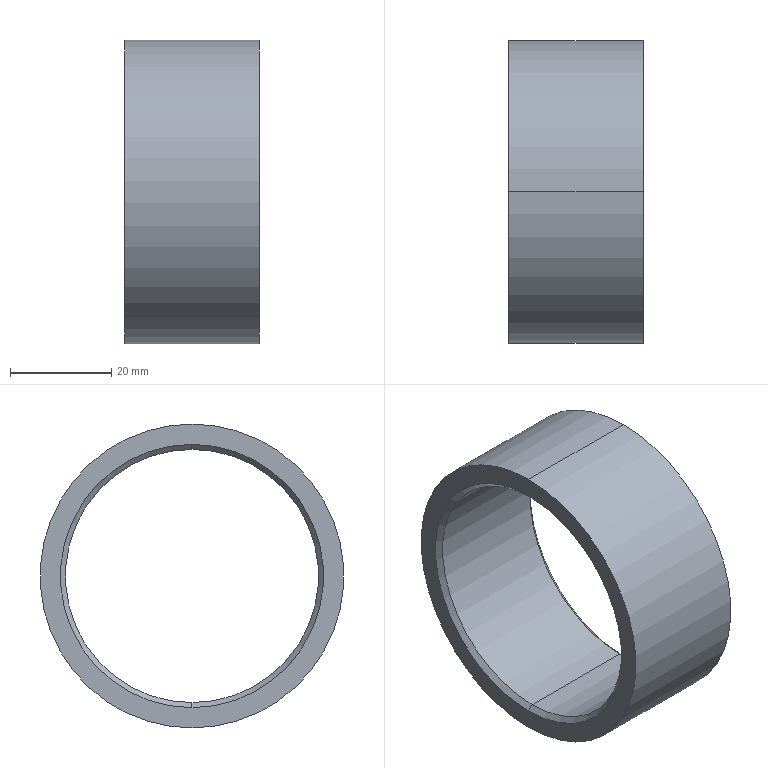Component | SolidWorks | SpindleSleeve4-1 | 1 solid | 10 faces | box 26.5 x 60 x 60 mm | volume 22735 mm3 | cone 4 | cylinder 4 | plane 2 | commonest cylinder face diameters 50 x2 60 x2
build123d program:
from build123d import *

# Parameters (mm, degrees)
SKETCH1_R           = 30
SKETCH1_R_2         = 25
BOSS_EXTRUDE1_DEPTH = 13.25
CHAMFER1_SIZE       = 1


with BuildPart() as part:
    # Sketch1 → Boss-Extrude1 (new, symmetric)
    with BuildSketch(Plane(origin=(0, 0, 0), x_dir=(0, 0, -1), z_dir=(1, 0, 0))):
        Circle(SKETCH1_R)
        Circle(SKETCH1_R_2, mode=Mode.SUBTRACT)
    extrude(amount=BOSS_EXTRUDE1_DEPTH, both=True)

    # Chamfer1
    chamfer1_edges = [part.edges().sort_by_distance(p)[0] for p in [
        (-13.25, 0, 25),
        (13.25, 0, 25),
    ]]
    chamfer(chamfer1_edges, length=CHAMFER1_SIZE)


solid = part.part

# Placed as in the assembly
solid = solid.moved(Location((-804.447, 34.532, 0), (0, 0, 0)))
STEP:
#1=COLOUR_RGB('',0.7922,0.8196,0.9333);
#2=FILL_AREA_STYLE_COLOUR('',#1);
#3=FILL_AREA_STYLE('',(#2));
#4=SURFACE_STYLE_FILL_AREA(#3);
#5=SURFACE_SIDE_STYLE('',(#4));
#6=SURFACE_STYLE_USAGE(.BOTH.,#5);
#7=PRESENTATION_STYLE_ASSIGNMENT((#6));
#8=CARTESIAN_POINT('',(-31.189,1.36,0.9843));
#9=VERTEX_POINT('',#8);
#10=CARTESIAN_POINT('',(-31.189,1.36,-0.9843));
#11=VERTEX_POINT('',#10);
#12=CARTESIAN_POINT('',(-31.189,1.36,0.));
#13=DIRECTION('',(1.,0.,0.));
#14=DIRECTION('',(0.,0.,-1.));
#15=AXIS2_PLACEMENT_3D('',#12,#13,#14);
#16=CIRCLE('',#15,0.9843);
#17=EDGE_CURVE('',#9,#11,#16,.T.);
#18=ORIENTED_EDGE('',*,*,#17,.F.);
#19=CARTESIAN_POINT('',(-31.149,1.36,1.024));
#20=VERTEX_POINT('',#19);
#21=CARTESIAN_POINT('',(-31.189,1.36,0.9843));
#22=DIRECTION('',(0.7071,0.,0.7071));
#23=VECTOR('',#22,39.37);
#24=LINE('',#21,#23);
#25=EDGE_CURVE('',#9,#20,#24,.T.);
#26=ORIENTED_EDGE('',*,*,#25,.T.);
#27=CARTESIAN_POINT('',(-31.149,1.36,-1.024));
#28=VERTEX_POINT('',#27);
#29=CARTESIAN_POINT('',(-31.149,1.36,0.));
#30=DIRECTION('',(-1.,0.,0.));
#31=DIRECTION('',(0.,0.,-1.));
#32=AXIS2_PLACEMENT_3D('',#29,#30,#31);
#33=CIRCLE('',#32,1.024);
#34=EDGE_CURVE('',#28,#20,#33,.T.);
#35=ORIENTED_EDGE('',*,*,#34,.F.);
#36=CARTESIAN_POINT('',(-31.189,1.36,-0.9843));
#37=DIRECTION('',(0.7071,0.,-0.7071));
#38=VECTOR('',#37,39.37);
#39=LINE('',#36,#38);
#40=EDGE_CURVE('',#11,#28,#39,.T.);
#41=ORIENTED_EDGE('',*,*,#40,.F.);
#42=EDGE_LOOP('',(#18,#26,#35,#41));
#43=FACE_OUTER_BOUND('',#42,.T.);
#44=CARTESIAN_POINT('',(-31.189,1.36,0.));
#45=DIRECTION('',(1.,0.,0.));
#46=DIRECTION('',(0.,0.,-1.));
#47=AXIS2_PLACEMENT_3D('',#44,#45,#46);
#48=CONICAL_SURFACE('',#47,0.9843,0.7854);
#49=ADVANCED_FACE('',(#43),#48,.F.);
#50=CARTESIAN_POINT('',(-32.153,1.36,-0.9843));
#51=VERTEX_POINT('',#50);
#52=CARTESIAN_POINT('',(-32.153,1.36,0.9843));
#53=VERTEX_POINT('',#52);
#54=CARTESIAN_POINT('',(-32.153,1.36,0.));
#55=DIRECTION('',(-1.,0.,0.));
#56=DIRECTION('',(0.,0.,-1.));
#57=AXIS2_PLACEMENT_3D('',#54,#55,#56);
#58=CIRCLE('',#57,0.9843);
#59=EDGE_CURVE('',#51,#53,#58,.T.);
#60=ORIENTED_EDGE('',*,*,#59,.F.);
#61=CARTESIAN_POINT('',(-32.193,1.36,-1.024));
#62=VERTEX_POINT('',#61);
#63=CARTESIAN_POINT('',(-32.193,1.36,-1.024));
#64=DIRECTION('',(-0.7071,0.,-0.7071));
#65=VECTOR('',#64,39.37);
#66=LINE('',#63,#65);
#67=EDGE_CURVE('',#51,#62,#66,.T.);
#68=ORIENTED_EDGE('',*,*,#67,.T.);
#69=CARTESIAN_POINT('',(-32.193,1.36,1.024));
#70=VERTEX_POINT('',#69);
#71=CARTESIAN_POINT('',(-32.193,1.36,0.));
#72=DIRECTION('',(1.,0.,0.));
#73=DIRECTION('',(0.,0.,-1.));
#74=AXIS2_PLACEMENT_3D('',#71,#72,#73);
#75=CIRCLE('',#74,1.024);
#76=EDGE_CURVE('',#70,#62,#75,.T.);
#77=ORIENTED_EDGE('',*,*,#76,.F.);
#78=CARTESIAN_POINT('',(-32.193,1.36,1.024));
#79=DIRECTION('',(-0.7071,0.,0.7071));
#80=VECTOR('',#79,39.37);
#81=LINE('',#78,#80);
#82=EDGE_CURVE('',#53,#70,#81,.T.);
#83=ORIENTED_EDGE('',*,*,#82,.F.);
#84=EDGE_LOOP('',(#60,#68,#77,#83));
#85=FACE_OUTER_BOUND('',#84,.T.);
#86=CARTESIAN_POINT('',(-32.193,1.36,0.));
#87=DIRECTION('',(-1.,0.,0.));
#88=DIRECTION('',(0.,0.,1.));
#89=AXIS2_PLACEMENT_3D('',#86,#87,#88);
#90=CONICAL_SURFACE('',#89,1.024,0.7854);
#91=ADVANCED_FACE('',(#85),#90,.F.);
#92=ORIENTED_EDGE('',*,*,#17,.T.);
#93=CARTESIAN_POINT('',(-31.149,1.36,-0.9843));
#94=DIRECTION('',(-1.,0.,0.));
#95=VECTOR('',#94,39.37);
#96=LINE('',#93,#95);
#97=EDGE_CURVE('',#11,#51,#96,.T.);
#98=ORIENTED_EDGE('',*,*,#97,.T.);
#99=ORIENTED_EDGE('',*,*,#59,.T.);
#100=CARTESIAN_POINT('',(-31.149,1.36,0.9843));
#101=DIRECTION('',(-1.,0.,0.));
#102=VECTOR('',#101,39.37);
#103=LINE('',#100,#102);
#104=EDGE_CURVE('',#9,#53,#103,.T.);
#105=ORIENTED_EDGE('',*,*,#104,.F.);
#106=EDGE_LOOP('',(#92,#98,#99,#105));
#107=FACE_OUTER_BOUND('',#106,.T.);
#108=CARTESIAN_POINT('',(-31.149,1.36,0.));
#109=DIRECTION('',(-1.,0.,0.));
#110=DIRECTION('',(0.,0.,1.));
#111=AXIS2_PLACEMENT_3D('',#108,#109,#110);
#112=CYLINDRICAL_SURFACE('',#111,0.9843);
#113=ADVANCED_FACE('',(#107),#112,.F.);
#114=CARTESIAN_POINT('',(-31.149,1.36,-1.181));
#115=VERTEX_POINT('',#114);
#116=CARTESIAN_POINT('',(-31.149,1.36,1.181));
#117=VERTEX_POINT('',#116);
#118=CARTESIAN_POINT('',(-31.149,1.36,0.));
#119=DIRECTION('',(1.,0.,0.));
#120=DIRECTION('',(0.,0.,-1.));
#121=AXIS2_PLACEMENT_3D('',#118,#119,#120);
#122=CIRCLE('',#121,1.181);
#123=EDGE_CURVE('',#115,#117,#122,.T.);
#124=ORIENTED_EDGE('',*,*,#123,.F.);
#125=CARTESIAN_POINT('',(-32.193,1.36,-1.181));
#126=VERTEX_POINT('',#125);
#127=CARTESIAN_POINT('',(-31.149,1.36,-1.181));
#128=DIRECTION('',(-1.,0.,0.));
#129=VECTOR('',#128,39.37);
#130=LINE('',#127,#129);
#131=EDGE_CURVE('',#115,#126,#130,.T.);
#132=ORIENTED_EDGE('',*,*,#131,.T.);
#133=CARTESIAN_POINT('',(-32.193,1.36,1.181));
#134=VERTEX_POINT('',#133);
#135=CARTESIAN_POINT('',(-32.193,1.36,0.));
#136=DIRECTION('',(1.,0.,0.));
#137=DIRECTION('',(0.,0.,-1.));
#138=AXIS2_PLACEMENT_3D('',#135,#136,#137);
#139=CIRCLE('',#138,1.181);
#140=EDGE_CURVE('',#126,#134,#139,.T.);
#141=ORIENTED_EDGE('',*,*,#140,.T.);
#142=CARTESIAN_POINT('',(-31.149,1.36,1.181));
#143=DIRECTION('',(-1.,0.,0.));
#144=VECTOR('',#143,39.37);
#145=LINE('',#142,#144);
#146=EDGE_CURVE('',#117,#134,#145,.T.);
#147=ORIENTED_EDGE('',*,*,#146,.F.);
#148=EDGE_LOOP('',(#124,#132,#141,#147));
#149=FACE_OUTER_BOUND('',#148,.T.);
#150=CARTESIAN_POINT('',(-31.149,1.36,0.));
#151=DIRECTION('',(-1.,0.,0.));
#152=DIRECTION('',(0.,0.,1.));
#153=AXIS2_PLACEMENT_3D('',#150,#151,#152);
#154=CYLINDRICAL_SURFACE('',#153,1.181);
#155=ADVANCED_FACE('',(#149),#154,.T.);
#156=ORIENTED_EDGE('',*,*,#34,.T.);
#157=CARTESIAN_POINT('',(-31.149,1.36,0.));
#158=DIRECTION('',(-1.,0.,0.));
#159=DIRECTION('',(0.,0.,-1.));
#160=AXIS2_PLACEMENT_3D('',#157,#158,#159);
#161=CIRCLE('',#160,1.024);
#162=EDGE_CURVE('',#20,#28,#161,.T.);
#163=ORIENTED_EDGE('',*,*,#162,.T.);
#164=EDGE_LOOP('',(#156,#163));
#165=FACE_BOUND('',#164,.T.);
#166=CARTESIAN_POINT('',(-31.149,1.36,0.));
#167=DIRECTION('',(1.,0.,0.));
#168=DIRECTION('',(0.,0.,-1.));
#169=AXIS2_PLACEMENT_3D('',#166,#167,#168);
#170=CIRCLE('',#169,1.181);
#171=EDGE_CURVE('',#117,#115,#170,.T.);
#172=ORIENTED_EDGE('',*,*,#171,.T.);
#173=ORIENTED_EDGE('',*,*,#123,.T.);
#174=EDGE_LOOP('',(#172,#173));
#175=FACE_OUTER_BOUND('',#174,.T.);
#176=CARTESIAN_POINT('',(-31.149,1.36,0.));
#177=DIRECTION('',(1.,0.,0.));
#178=DIRECTION('',(0.,0.,-1.));
#179=AXIS2_PLACEMENT_3D('',#176,#177,#178);
#180=PLANE('',#179);
#181=ADVANCED_FACE('',(#165,#175),#180,.T.);
#182=ORIENTED_EDGE('',*,*,#76,.T.);
#183=CARTESIAN_POINT('',(-32.193,1.36,0.));
#184=DIRECTION('',(1.,0.,0.));
#185=DIRECTION('',(0.,0.,-1.));
#186=AXIS2_PLACEMENT_3D('',#183,#184,#185);
#187=CIRCLE('',#186,1.024);
#188=EDGE_CURVE('',#62,#70,#187,.T.);
#189=ORIENTED_EDGE('',*,*,#188,.T.);
#190=EDGE_LOOP('',(#182,#189));
#191=FACE_BOUND('',#190,.T.);
#192=CARTESIAN_POINT('',(-32.193,1.36,0.));
#193=DIRECTION('',(1.,0.,0.));
#194=DIRECTION('',(0.,0.,-1.));
#195=AXIS2_PLACEMENT_3D('',#192,#193,#194);
#196=CIRCLE('',#195,1.181);
#197=EDGE_CURVE('',#134,#126,#196,.T.);
#198=ORIENTED_EDGE('',*,*,#197,.F.);
#199=ORIENTED_EDGE('',*,*,#140,.F.);
#200=EDGE_LOOP('',(#198,#199));
#201=FACE_OUTER_BOUND('',#200,.T.);
#202=CARTESIAN_POINT('',(-32.193,1.36,0.));
#203=DIRECTION('',(1.,0.,0.));
#204=DIRECTION('',(0.,0.,-1.));
#205=AXIS2_PLACEMENT_3D('',#202,#203,#204);
#206=PLANE('',#205);
#207=ADVANCED_FACE('',(#191,#201),#206,.F.);
#208=ORIENTED_EDGE('',*,*,#131,.F.);
#209=ORIENTED_EDGE('',*,*,#171,.F.);
#210=ORIENTED_EDGE('',*,*,#146,.T.);
#211=ORIENTED_EDGE('',*,*,#197,.T.);
#212=EDGE_LOOP('',(#208,#209,#210,#211));
#213=FACE_OUTER_BOUND('',#212,.T.);
#214=CARTESIAN_POINT('',(-31.149,1.36,0.));
#215=DIRECTION('',(-1.,0.,0.));
#216=DIRECTION('',(0.,0.,1.));
#217=AXIS2_PLACEMENT_3D('',#214,#215,#216);
#218=CYLINDRICAL_SURFACE('',#217,1.181);
#219=ADVANCED_FACE('',(#213),#218,.T.);
#220=ORIENTED_EDGE('',*,*,#97,.F.);
#221=CARTESIAN_POINT('',(-31.189,1.36,0.));
#222=DIRECTION('',(1.,0.,0.));
#223=DIRECTION('',(0.,0.,-1.));
#224=AXIS2_PLACEMENT_3D('',#221,#222,#223);
#225=CIRCLE('',#224,0.9843);
#226=EDGE_CURVE('',#11,#9,#225,.T.);
#227=ORIENTED_EDGE('',*,*,#226,.T.);
#228=ORIENTED_EDGE('',*,*,#104,.T.);
#229=CARTESIAN_POINT('',(-32.153,1.36,0.));
#230=DIRECTION('',(-1.,0.,0.));
#231=DIRECTION('',(0.,0.,-1.));
#232=AXIS2_PLACEMENT_3D('',#229,#230,#231);
#233=CIRCLE('',#232,0.9843);
#234=EDGE_CURVE('',#53,#51,#233,.T.);
#235=ORIENTED_EDGE('',*,*,#234,.T.);
#236=EDGE_LOOP('',(#220,#227,#228,#235));
#237=FACE_OUTER_BOUND('',#236,.T.);
#238=CARTESIAN_POINT('',(-31.149,1.36,0.));
#239=DIRECTION('',(-1.,0.,0.));
#240=DIRECTION('',(0.,0.,1.));
#241=AXIS2_PLACEMENT_3D('',#238,#239,#240);
#242=CYLINDRICAL_SURFACE('',#241,0.9843);
#243=ADVANCED_FACE('',(#237),#242,.F.);
#244=ORIENTED_EDGE('',*,*,#67,.F.);
#245=ORIENTED_EDGE('',*,*,#234,.F.);
#246=ORIENTED_EDGE('',*,*,#82,.T.);
#247=ORIENTED_EDGE('',*,*,#188,.F.);
#248=EDGE_LOOP('',(#244,#245,#246,#247));
#249=FACE_OUTER_BOUND('',#248,.T.);
#250=CARTESIAN_POINT('',(-32.193,1.36,0.));
#251=DIRECTION('',(-1.,0.,0.));
#252=DIRECTION('',(0.,0.,1.));
#253=AXIS2_PLACEMENT_3D('',#250,#251,#252);
#254=CONICAL_SURFACE('',#253,1.024,0.7854);
#255=ADVANCED_FACE('',(#249),#254,.F.);
#256=ORIENTED_EDGE('',*,*,#25,.F.);
#257=ORIENTED_EDGE('',*,*,#226,.F.);
#258=ORIENTED_EDGE('',*,*,#40,.T.);
#259=ORIENTED_EDGE('',*,*,#162,.F.);
#260=EDGE_LOOP('',(#256,#257,#258,#259));
#261=FACE_OUTER_BOUND('',#260,.T.);
#262=CARTESIAN_POINT('',(-31.189,1.36,0.));
#263=DIRECTION('',(1.,0.,0.));
#264=DIRECTION('',(0.,0.,-1.));
#265=AXIS2_PLACEMENT_3D('',#262,#263,#264);
#266=CONICAL_SURFACE('',#265,0.9843,0.7854);
#267=ADVANCED_FACE('',(#261),#266,.F.);
#268=CLOSED_SHELL('',(#49,#91,#113,#155,#181,#207,#219,#243,#255,#267));
#269=MANIFOLD_SOLID_BREP('',#268);
#270=STYLED_ITEM('',(#7),#269);
#271=PRESENTATION_LAYER_ASSIGNMENT('','',(#270));
#272=(LENGTH_UNIT()NAMED_UNIT(*)SI_UNIT($,.METRE.));
#273=LENGTH_MEASURE_WITH_UNIT(LENGTH_MEASURE(0.0254),#272);
#274=DIMENSIONAL_EXPONENTS(1.,0.,0.,0.,0.,0.,0.);
#275=(CONVERSION_BASED_UNIT('',#273)LENGTH_UNIT()NAMED_UNIT(#274));
#276=UNCERTAINTY_MEASURE_WITH_UNIT(LENGTH_MEASURE(0.00001),#275,'','');
#277=(NAMED_UNIT(*)PLANE_ANGLE_UNIT()SI_UNIT($,.RADIAN.));
#278=(NAMED_UNIT(*)SI_UNIT($,.STERADIAN.)SOLID_ANGLE_UNIT());
#279=(GEOMETRIC_REPRESENTATION_CONTEXT(3)GLOBAL_UNCERTAINTY_ASSIGNED_CONTEXT((#276))GLOBAL_UNIT_ASSIGNED_CONTEXT((#275,#277,#278))REPRESENTATION_CONTEXT('',''));
#280=MECHANICAL_DESIGN_GEOMETRIC_PRESENTATION_REPRESENTATION('',(#270),#279);
#281=CARTESIAN_POINT('',(0.,0.,0.));
#282=DIRECTION('',(0.,0.,1.));
#283=DIRECTION('',(1.,0.,0.));
#284=AXIS2_PLACEMENT_3D('',#281,#282,#283);
#285=(LENGTH_UNIT()NAMED_UNIT(*)SI_UNIT($,.METRE.));
#286=LENGTH_MEASURE_WITH_UNIT(LENGTH_MEASURE(0.0254),#285);
#287=DIMENSIONAL_EXPONENTS(1.,0.,0.,0.,0.,0.,0.);
#288=(CONVERSION_BASED_UNIT('',#286)LENGTH_UNIT()NAMED_UNIT(#287));
#289=UNCERTAINTY_MEASURE_WITH_UNIT(LENGTH_MEASURE(0.00001),#288,'','');
#290=(NAMED_UNIT(*)PLANE_ANGLE_UNIT()SI_UNIT($,.RADIAN.));
#291=(NAMED_UNIT(*)SI_UNIT($,.STERADIAN.)SOLID_ANGLE_UNIT());
#292=(GEOMETRIC_REPRESENTATION_CONTEXT(3)GLOBAL_UNCERTAINTY_ASSIGNED_CONTEXT((#289))GLOBAL_UNIT_ASSIGNED_CONTEXT((#288,#290,#291))REPRESENTATION_CONTEXT('',''));
#293=ADVANCED_BREP_SHAPE_REPRESENTATION('',(#269,#284),#292);